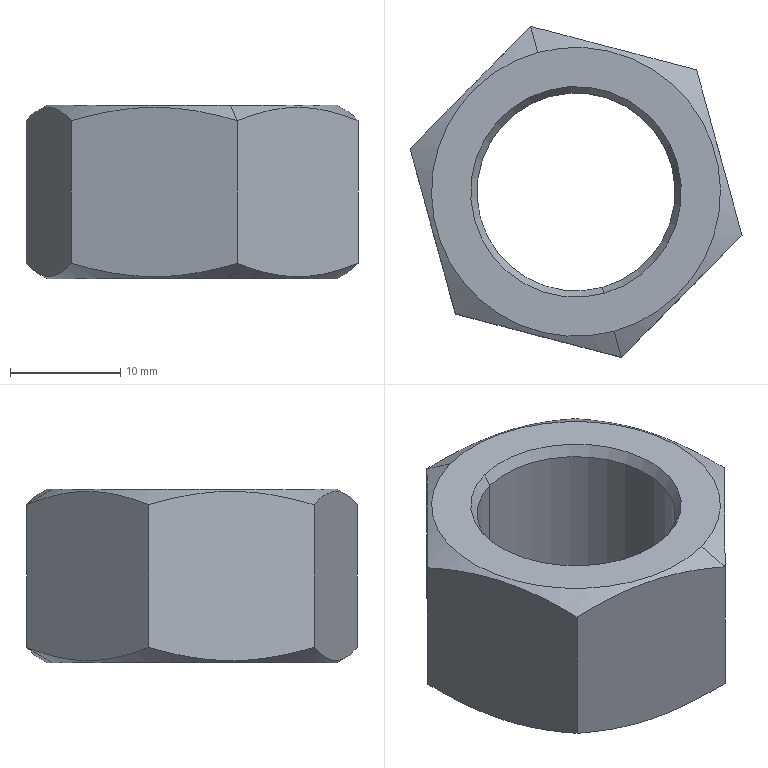Component | SolidWorks | Cylinder-1_hex nuts 1-fine pitch-grades ab gb-9 | 1 solid | 18 faces | box 30.16 x 30.07 x 15.8 mm | volume 5847 mm3 | cone 8 | plane 8 | cylinder 2 | commonest cylinder face diameters 18 x2
STEP:
#1=COLOUR_RGB('',0.7922,0.8196,0.9333);
#2=FILL_AREA_STYLE_COLOUR('',#1);
#3=FILL_AREA_STYLE('',(#2));
#4=SURFACE_STYLE_FILL_AREA(#3);
#5=SURFACE_SIDE_STYLE('',(#4));
#6=SURFACE_STYLE_USAGE(.BOTH.,#5);
#7=PRESENTATION_STYLE_ASSIGNMENT((#6));
#8=CARTESIAN_POINT('',(-7.202,1.382,-13.665));
#9=VERTEX_POINT('',#8);
#10=CARTESIAN_POINT('',(-7.015,0.6981,-13.665));
#11=VERTEX_POINT('',#10);
#12=CARTESIAN_POINT('',(-7.109,1.04,-13.665));
#13=DIRECTION('',(0.,-0.,-1.));
#14=DIRECTION('',(-0.2645,0.9644,0.));
#15=AXIS2_PLACEMENT_3D('',#12,#13,#14);
#16=CIRCLE('',#15,0.3543);
#17=EDGE_CURVE('',#9,#11,#16,.T.);
#18=ORIENTED_EDGE('',*,*,#17,.F.);
#19=CARTESIAN_POINT('',(-7.213,1.419,-13.687));
#20=VERTEX_POINT('',#19);
#21=CARTESIAN_POINT('',(-7.202,1.382,-13.665));
#22=DIRECTION('',(-0.2291,0.8352,-0.5));
#23=VECTOR('',#22,39.37);
#24=LINE('',#21,#23);
#25=EDGE_CURVE('',#9,#20,#24,.T.);
#26=ORIENTED_EDGE('',*,*,#25,.T.);
#27=CARTESIAN_POINT('',(-7.005,0.6606,-13.687));
#28=VERTEX_POINT('',#27);
#29=CARTESIAN_POINT('',(-7.109,1.04,-13.687));
#30=DIRECTION('',(-0.,0.,1.));
#31=DIRECTION('',(-0.2645,0.9644,0.));
#32=AXIS2_PLACEMENT_3D('',#29,#30,#31);
#33=CIRCLE('',#32,0.3932);
#34=EDGE_CURVE('',#28,#20,#33,.T.);
#35=ORIENTED_EDGE('',*,*,#34,.F.);
#36=CARTESIAN_POINT('',(-7.015,0.6981,-13.665));
#37=DIRECTION('',(0.2291,-0.8352,-0.5));
#38=VECTOR('',#37,39.37);
#39=LINE('',#36,#38);
#40=EDGE_CURVE('',#11,#28,#39,.T.);
#41=ORIENTED_EDGE('',*,*,#40,.F.);
#42=EDGE_LOOP('',(#18,#26,#35,#41));
#43=FACE_OUTER_BOUND('',#42,.T.);
#44=CARTESIAN_POINT('',(-7.109,1.04,-13.665));
#45=DIRECTION('',(0.,-0.,-1.));
#46=DIRECTION('',(0.2645,-0.9644,0.));
#47=AXIS2_PLACEMENT_3D('',#44,#45,#46);
#48=CONICAL_SURFACE('',#47,0.3543,1.047);
#49=ADVANCED_FACE('',(#43),#48,.F.);
#50=CARTESIAN_POINT('',(-7.015,0.6981,-13.104));
#51=VERTEX_POINT('',#50);
#52=CARTESIAN_POINT('',(-7.202,1.382,-13.104));
#53=VERTEX_POINT('',#52);
#54=CARTESIAN_POINT('',(-7.109,1.04,-13.104));
#55=DIRECTION('',(-0.,0.,1.));
#56=DIRECTION('',(-0.2645,0.9644,0.));
#57=AXIS2_PLACEMENT_3D('',#54,#55,#56);
#58=CIRCLE('',#57,0.3543);
#59=EDGE_CURVE('',#51,#53,#58,.T.);
#60=ORIENTED_EDGE('',*,*,#59,.F.);
#61=CARTESIAN_POINT('',(-7.009,0.6765,-13.065));
#62=VERTEX_POINT('',#61);
#63=CARTESIAN_POINT('',(-7.009,0.6765,-13.065));
#64=DIRECTION('',(0.1323,-0.4822,0.866));
#65=VECTOR('',#64,39.37);
#66=LINE('',#63,#65);
#67=EDGE_CURVE('',#51,#62,#66,.T.);
#68=ORIENTED_EDGE('',*,*,#67,.T.);
#69=CARTESIAN_POINT('',(-7.208,1.403,-13.065));
#70=VERTEX_POINT('',#69);
#71=CARTESIAN_POINT('',(-7.109,1.04,-13.065));
#72=DIRECTION('',(0.,-0.,-1.));
#73=DIRECTION('',(-0.2645,0.9644,0.));
#74=AXIS2_PLACEMENT_3D('',#71,#72,#73);
#75=CIRCLE('',#74,0.3768);
#76=EDGE_CURVE('',#70,#62,#75,.T.);
#77=ORIENTED_EDGE('',*,*,#76,.F.);
#78=CARTESIAN_POINT('',(-7.208,1.403,-13.065));
#79=DIRECTION('',(-0.1323,0.4822,0.866));
#80=VECTOR('',#79,39.37);
#81=LINE('',#78,#80);
#82=EDGE_CURVE('',#53,#70,#81,.T.);
#83=ORIENTED_EDGE('',*,*,#82,.F.);
#84=EDGE_LOOP('',(#60,#68,#77,#83));
#85=FACE_OUTER_BOUND('',#84,.T.);
#86=CARTESIAN_POINT('',(-7.109,1.04,-13.065));
#87=DIRECTION('',(-0.,0.,1.));
#88=DIRECTION('',(-0.2645,0.9644,0.));
#89=AXIS2_PLACEMENT_3D('',#86,#87,#88);
#90=CONICAL_SURFACE('',#89,0.3768,0.5236);
#91=ADVANCED_FACE('',(#85),#90,.F.);
#92=CARTESIAN_POINT('',(-7.245,1.538,-13.687));
#93=VERTEX_POINT('',#92);
#94=CARTESIAN_POINT('',(-6.972,0.5415,-13.687));
#95=VERTEX_POINT('',#94);
#96=CARTESIAN_POINT('',(-7.109,1.04,-13.687));
#97=DIRECTION('',(0.,0.,1.));
#98=DIRECTION('',(-0.2645,0.9644,0.));
#99=AXIS2_PLACEMENT_3D('',#96,#97,#98);
#100=CIRCLE('',#99,0.5167);
#101=EDGE_CURVE('',#93,#95,#100,.T.);
#102=ORIENTED_EDGE('',*,*,#101,.T.);
#103=CARTESIAN_POINT('',(-6.946,0.448,-13.631));
#104=VERTEX_POINT('',#103);
#105=CARTESIAN_POINT('',(-6.972,0.5415,-13.687));
#106=DIRECTION('',(0.2291,-0.8352,0.5));
#107=VECTOR('',#106,39.37);
#108=LINE('',#105,#107);
#109=EDGE_CURVE('',#95,#104,#108,.T.);
#110=ORIENTED_EDGE('',*,*,#109,.T.);
#111=CARTESIAN_POINT('',(-7.54,0.6033,-13.631));
#112=VERTEX_POINT('',#111);
#113=CARTESIAN_POINT('',(-6.946,0.448,-13.631));
#114=CARTESIAN_POINT('',(-6.995,0.4607,-13.646));
#115=CARTESIAN_POINT('',(-7.043,0.4734,-13.657));
#116=CARTESIAN_POINT('',(-7.142,0.4993,-13.674));
#117=CARTESIAN_POINT('',(-7.192,0.5123,-13.678));
#118=CARTESIAN_POINT('',(-7.268,0.5321,-13.679));
#119=CARTESIAN_POINT('',(-7.293,0.5387,-13.677));
#120=CARTESIAN_POINT('',(-7.343,0.5519,-13.673));
#121=CARTESIAN_POINT('',(-7.368,0.5584,-13.67));
#122=CARTESIAN_POINT('',(-7.442,0.5778,-13.657));
#123=CARTESIAN_POINT('',(-7.491,0.5906,-13.646));
#124=CARTESIAN_POINT('',(-7.54,0.6033,-13.631));
#125=B_SPLINE_CURVE_WITH_KNOTS('',3,(#113,#114,#115,#116,#117,#118,#119,#120,#121,#122,#123,#124),.UNSPECIFIED.,.F.,.F.,(4,2,2,2,2,4),(0.00000024,0.003936,0.007872,0.00984,0.01181,0.01574),.UNSPECIFIED.);
#126=EDGE_CURVE('',#104,#112,#125,.T.);
#127=ORIENTED_EDGE('',*,*,#126,.T.);
#128=CARTESIAN_POINT('',(-7.702,1.195,-13.631));
#129=VERTEX_POINT('',#128);
#130=CARTESIAN_POINT('',(-7.54,0.6033,-13.631));
#131=CARTESIAN_POINT('',(-7.553,0.6511,-13.645));
#132=CARTESIAN_POINT('',(-7.566,0.6996,-13.657));
#133=CARTESIAN_POINT('',(-7.587,0.7737,-13.67));
#134=CARTESIAN_POINT('',(-7.594,0.7987,-13.673));
#135=CARTESIAN_POINT('',(-7.607,0.8491,-13.677));
#136=CARTESIAN_POINT('',(-7.614,0.8741,-13.679));
#137=CARTESIAN_POINT('',(-7.635,0.9492,-13.679));
#138=CARTESIAN_POINT('',(-7.648,0.9989,-13.674));
#139=CARTESIAN_POINT('',(-7.669,1.073,-13.662));
#140=CARTESIAN_POINT('',(-7.676,1.098,-13.657));
#141=CARTESIAN_POINT('',(-7.689,1.147,-13.645));
#142=CARTESIAN_POINT('',(-7.696,1.171,-13.638));
#143=CARTESIAN_POINT('',(-7.702,1.195,-13.631));
#144=B_SPLINE_CURVE_WITH_KNOTS('',3,(#130,#131,#132,#133,#134,#135,#136,#137,#138,#139,#140,#141,#142,#143),.UNSPECIFIED.,.F.,.F.,(4,2,2,2,2,2,4),(0.005749,0.009683,0.01165,0.01362,0.01755,0.01952,0.02148),.UNSPECIFIED.);
#145=EDGE_CURVE('',#112,#129,#144,.T.);
#146=ORIENTED_EDGE('',*,*,#145,.T.);
#147=CARTESIAN_POINT('',(-7.271,1.632,-13.631));
#148=VERTEX_POINT('',#147);
#149=CARTESIAN_POINT('',(-7.702,1.195,-13.631));
#150=CARTESIAN_POINT('',(-7.667,1.231,-13.646));
#151=CARTESIAN_POINT('',(-7.632,1.267,-13.657));
#152=CARTESIAN_POINT('',(-7.56,1.339,-13.674));
#153=CARTESIAN_POINT('',(-7.524,1.376,-13.678));
#154=CARTESIAN_POINT('',(-7.469,1.432,-13.679));
#155=CARTESIAN_POINT('',(-7.45,1.45,-13.677));
#156=CARTESIAN_POINT('',(-7.414,1.487,-13.673));
#157=CARTESIAN_POINT('',(-7.396,1.505,-13.67));
#158=CARTESIAN_POINT('',(-7.342,1.56,-13.657));
#159=CARTESIAN_POINT('',(-7.306,1.596,-13.646));
#160=CARTESIAN_POINT('',(-7.271,1.632,-13.631));
#161=B_SPLINE_CURVE_WITH_KNOTS('',3,(#149,#150,#151,#152,#153,#154,#155,#156,#157,#158,#159,#160),.UNSPECIFIED.,.F.,.F.,(4,2,2,2,2,4),(0.00000024,0.003936,0.007872,0.00984,0.01181,0.01574),.UNSPECIFIED.);
#162=EDGE_CURVE('',#129,#148,#161,.T.);
#163=ORIENTED_EDGE('',*,*,#162,.T.);
#164=CARTESIAN_POINT('',(-7.245,1.538,-13.687));
#165=DIRECTION('',(-0.2291,0.8352,0.5));
#166=VECTOR('',#165,39.37);
#167=LINE('',#164,#166);
#168=EDGE_CURVE('',#93,#148,#167,.T.);
#169=ORIENTED_EDGE('',*,*,#168,.F.);
#170=EDGE_LOOP('',(#102,#110,#127,#146,#163,#169));
#171=FACE_OUTER_BOUND('',#170,.T.);
#172=CARTESIAN_POINT('',(-7.109,1.04,-13.687));
#173=DIRECTION('',(0.,0.,1.));
#174=DIRECTION('',(-0.2645,0.9644,0.));
#175=AXIS2_PLACEMENT_3D('',#172,#173,#174);
#176=CONICAL_SURFACE('',#175,0.5167,1.047);
#177=ADVANCED_FACE('',(#171),#176,.T.);
#178=CARTESIAN_POINT('',(-7.245,1.538,-13.065));
#179=VERTEX_POINT('',#178);
#180=CARTESIAN_POINT('',(-6.972,0.5415,-13.065));
#181=VERTEX_POINT('',#180);
#182=CARTESIAN_POINT('',(-7.109,1.04,-13.065));
#183=DIRECTION('',(0.,0.,1.));
#184=DIRECTION('',(-0.2645,0.9644,0.));
#185=AXIS2_PLACEMENT_3D('',#182,#183,#184);
#186=CIRCLE('',#185,0.5167);
#187=EDGE_CURVE('',#179,#181,#186,.T.);
#188=ORIENTED_EDGE('',*,*,#187,.F.);
#189=CARTESIAN_POINT('',(-7.271,1.632,-13.121));
#190=VERTEX_POINT('',#189);
#191=CARTESIAN_POINT('',(-7.271,1.632,-13.121));
#192=DIRECTION('',(-0.2291,0.8352,-0.5));
#193=VECTOR('',#192,39.37);
#194=LINE('',#191,#193);
#195=EDGE_CURVE('',#179,#190,#194,.T.);
#196=ORIENTED_EDGE('',*,*,#195,.T.);
#197=CARTESIAN_POINT('',(-7.702,1.195,-13.121));
#198=VERTEX_POINT('',#197);
#199=CARTESIAN_POINT('',(-7.271,1.632,-13.121));
#200=CARTESIAN_POINT('',(-7.306,1.596,-13.107));
#201=CARTESIAN_POINT('',(-7.342,1.56,-13.095));
#202=CARTESIAN_POINT('',(-7.413,1.488,-13.078));
#203=CARTESIAN_POINT('',(-7.449,1.451,-13.074));
#204=CARTESIAN_POINT('',(-7.505,1.395,-13.074));
#205=CARTESIAN_POINT('',(-7.523,1.377,-13.075));
#206=CARTESIAN_POINT('',(-7.559,1.34,-13.079));
#207=CARTESIAN_POINT('',(-7.577,1.321,-13.082));
#208=CARTESIAN_POINT('',(-7.631,1.267,-13.095));
#209=CARTESIAN_POINT('',(-7.667,1.231,-13.107));
#210=CARTESIAN_POINT('',(-7.702,1.195,-13.121));
#211=B_SPLINE_CURVE_WITH_KNOTS('',3,(#199,#200,#201,#202,#203,#204,#205,#206,#207,#208,#209,#210),.UNSPECIFIED.,.F.,.F.,(4,2,2,2,2,4),(0.00000024,0.003936,0.007872,0.00984,0.01181,0.01574),.UNSPECIFIED.);
#212=EDGE_CURVE('',#190,#198,#211,.T.);
#213=ORIENTED_EDGE('',*,*,#212,.T.);
#214=CARTESIAN_POINT('',(-7.54,0.6033,-13.121));
#215=VERTEX_POINT('',#214);
#216=CARTESIAN_POINT('',(-7.702,1.195,-13.121));
#217=CARTESIAN_POINT('',(-7.696,1.171,-13.114));
#218=CARTESIAN_POINT('',(-7.689,1.147,-13.107));
#219=CARTESIAN_POINT('',(-7.676,1.098,-13.095));
#220=CARTESIAN_POINT('',(-7.669,1.073,-13.09));
#221=CARTESIAN_POINT('',(-7.648,0.9989,-13.078));
#222=CARTESIAN_POINT('',(-7.635,0.9492,-13.074));
#223=CARTESIAN_POINT('',(-7.614,0.8741,-13.074));
#224=CARTESIAN_POINT('',(-7.607,0.8491,-13.075));
#225=CARTESIAN_POINT('',(-7.594,0.7987,-13.079));
#226=CARTESIAN_POINT('',(-7.587,0.7737,-13.082));
#227=CARTESIAN_POINT('',(-7.566,0.6996,-13.095));
#228=CARTESIAN_POINT('',(-7.553,0.6511,-13.107));
#229=CARTESIAN_POINT('',(-7.54,0.6033,-13.121));
#230=B_SPLINE_CURVE_WITH_KNOTS('',3,(#216,#217,#218,#219,#220,#221,#222,#223,#224,#225,#226,#227,#228,#229),.UNSPECIFIED.,.F.,.F.,(4,2,2,2,2,2,4),(0.01387,0.01584,0.01782,0.02176,0.02373,0.0257,0.02965),.UNSPECIFIED.);
#231=EDGE_CURVE('',#198,#215,#230,.T.);
#232=ORIENTED_EDGE('',*,*,#231,.T.);
#233=CARTESIAN_POINT('',(-6.946,0.448,-13.121));
#234=VERTEX_POINT('',#233);
#235=CARTESIAN_POINT('',(-7.54,0.6033,-13.121));
#236=CARTESIAN_POINT('',(-7.491,0.5906,-13.107));
#237=CARTESIAN_POINT('',(-7.443,0.5779,-13.095));
#238=CARTESIAN_POINT('',(-7.344,0.552,-13.078));
#239=CARTESIAN_POINT('',(-7.294,0.539,-13.074));
#240=CARTESIAN_POINT('',(-7.218,0.5192,-13.074));
#241=CARTESIAN_POINT('',(-7.193,0.5126,-13.075));
#242=CARTESIAN_POINT('',(-7.143,0.4994,-13.079));
#243=CARTESIAN_POINT('',(-7.118,0.4929,-13.082));
#244=CARTESIAN_POINT('',(-7.044,0.4735,-13.095));
#245=CARTESIAN_POINT('',(-6.995,0.4607,-13.107));
#246=CARTESIAN_POINT('',(-6.946,0.448,-13.121));
#247=B_SPLINE_CURVE_WITH_KNOTS('',3,(#235,#236,#237,#238,#239,#240,#241,#242,#243,#244,#245,#246),.UNSPECIFIED.,.F.,.F.,(4,2,2,2,2,4),(0.00000024,0.003936,0.007872,0.00984,0.01181,0.01574),.UNSPECIFIED.);
#248=EDGE_CURVE('',#215,#234,#247,.T.);
#249=ORIENTED_EDGE('',*,*,#248,.T.);
#250=CARTESIAN_POINT('',(-6.946,0.448,-13.121));
#251=DIRECTION('',(0.2291,-0.8352,-0.5));
#252=VECTOR('',#251,39.37);
#253=LINE('',#250,#252);
#254=EDGE_CURVE('',#181,#234,#253,.T.);
#255=ORIENTED_EDGE('',*,*,#254,.F.);
#256=EDGE_LOOP('',(#188,#196,#213,#232,#249,#255));
#257=FACE_OUTER_BOUND('',#256,.T.);
#258=CARTESIAN_POINT('',(-7.109,1.04,-13.121));
#259=DIRECTION('',(-0.,-0.,-1.));
#260=DIRECTION('',(0.2645,-0.9644,0.));
#261=AXIS2_PLACEMENT_3D('',#258,#259,#260);
#262=CONICAL_SURFACE('',#261,0.6137,1.047);
#263=ADVANCED_FACE('',(#257),#262,.T.);
#264=ORIENTED_EDGE('',*,*,#59,.T.);
#265=CARTESIAN_POINT('',(-7.202,1.382,-13.065));
#266=DIRECTION('',(0.,-0.,-1.));
#267=VECTOR('',#266,39.37);
#268=LINE('',#265,#267);
#269=EDGE_CURVE('',#53,#9,#268,.T.);
#270=ORIENTED_EDGE('',*,*,#269,.T.);
#271=ORIENTED_EDGE('',*,*,#17,.T.);
#272=CARTESIAN_POINT('',(-7.015,0.6981,-13.065));
#273=DIRECTION('',(0.,-0.,-1.));
#274=VECTOR('',#273,39.37);
#275=LINE('',#272,#274);
#276=EDGE_CURVE('',#51,#11,#275,.T.);
#277=ORIENTED_EDGE('',*,*,#276,.F.);
#278=EDGE_LOOP('',(#264,#270,#271,#277));
#279=FACE_OUTER_BOUND('',#278,.T.);
#280=CARTESIAN_POINT('',(-7.109,1.04,-13.065));
#281=DIRECTION('',(0.,-0.,-1.));
#282=DIRECTION('',(0.2645,-0.9644,0.));
#283=AXIS2_PLACEMENT_3D('',#280,#281,#282);
#284=CYLINDRICAL_SURFACE('',#283,0.3543);
#285=ADVANCED_FACE('',(#279),#284,.F.);
#286=CARTESIAN_POINT('',(-6.677,1.476,-13.631));
#287=VERTEX_POINT('',#286);
#288=CARTESIAN_POINT('',(-6.515,0.8845,-13.631));
#289=VERTEX_POINT('',#288);
#290=CARTESIAN_POINT('',(-6.677,1.476,-13.631));
#291=CARTESIAN_POINT('',(-6.671,1.452,-13.638));
#292=CARTESIAN_POINT('',(-6.664,1.428,-13.645));
#293=CARTESIAN_POINT('',(-6.65,1.379,-13.657));
#294=CARTESIAN_POINT('',(-6.644,1.354,-13.662));
#295=CARTESIAN_POINT('',(-6.623,1.28,-13.674));
#296=CARTESIAN_POINT('',(-6.61,1.23,-13.679));
#297=CARTESIAN_POINT('',(-6.589,1.155,-13.679));
#298=CARTESIAN_POINT('',(-6.582,1.13,-13.677));
#299=CARTESIAN_POINT('',(-6.568,1.08,-13.673));
#300=CARTESIAN_POINT('',(-6.562,1.055,-13.67));
#301=CARTESIAN_POINT('',(-6.541,0.9808,-13.657));
#302=CARTESIAN_POINT('',(-6.528,0.9323,-13.645));
#303=CARTESIAN_POINT('',(-6.515,0.8845,-13.631));
#304=B_SPLINE_CURVE_WITH_KNOTS('',3,(#290,#291,#292,#293,#294,#295,#296,#297,#298,#299,#300,#301,#302,#303),.UNSPECIFIED.,.F.,.F.,(4,2,2,2,2,2,4),(0.01387,0.01584,0.01782,0.02176,0.02373,0.0257,0.02965),.UNSPECIFIED.);
#305=EDGE_CURVE('',#287,#289,#304,.T.);
#306=ORIENTED_EDGE('',*,*,#305,.F.);
#307=CARTESIAN_POINT('',(-6.677,1.476,-13.121));
#308=VERTEX_POINT('',#307);
#309=CARTESIAN_POINT('',(-6.677,1.476,-13.065));
#310=DIRECTION('',(0.,-0.,-1.));
#311=VECTOR('',#310,39.37);
#312=LINE('',#309,#311);
#313=EDGE_CURVE('',#308,#287,#312,.T.);
#314=ORIENTED_EDGE('',*,*,#313,.F.);
#315=CARTESIAN_POINT('',(-6.515,0.8845,-13.121));
#316=VERTEX_POINT('',#315);
#317=CARTESIAN_POINT('',(-6.515,0.8845,-13.121));
#318=CARTESIAN_POINT('',(-6.528,0.9323,-13.107));
#319=CARTESIAN_POINT('',(-6.541,0.9808,-13.095));
#320=CARTESIAN_POINT('',(-6.562,1.055,-13.082));
#321=CARTESIAN_POINT('',(-6.568,1.08,-13.079));
#322=CARTESIAN_POINT('',(-6.582,1.13,-13.075));
#323=CARTESIAN_POINT('',(-6.589,1.155,-13.074));
#324=CARTESIAN_POINT('',(-6.61,1.23,-13.074));
#325=CARTESIAN_POINT('',(-6.623,1.28,-13.078));
#326=CARTESIAN_POINT('',(-6.644,1.354,-13.09));
#327=CARTESIAN_POINT('',(-6.65,1.379,-13.095));
#328=CARTESIAN_POINT('',(-6.664,1.428,-13.107));
#329=CARTESIAN_POINT('',(-6.671,1.452,-13.114));
#330=CARTESIAN_POINT('',(-6.677,1.476,-13.121));
#331=B_SPLINE_CURVE_WITH_KNOTS('',3,(#317,#318,#319,#320,#321,#322,#323,#324,#325,#326,#327,#328,#329,#330),.UNSPECIFIED.,.F.,.F.,(4,2,2,2,2,2,4),(0.005749,0.009683,0.01165,0.01362,0.01755,0.01952,0.02148),.UNSPECIFIED.);
#332=EDGE_CURVE('',#316,#308,#331,.T.);
#333=ORIENTED_EDGE('',*,*,#332,.F.);
#334=CARTESIAN_POINT('',(-6.515,0.8845,-13.065));
#335=DIRECTION('',(0.,-0.,-1.));
#336=VECTOR('',#335,39.37);
#337=LINE('',#334,#336);
#338=EDGE_CURVE('',#316,#289,#337,.T.);
#339=ORIENTED_EDGE('',*,*,#338,.T.);
#340=EDGE_LOOP('',(#306,#314,#333,#339));
#341=FACE_OUTER_BOUND('',#340,.T.);
#342=CARTESIAN_POINT('',(-6.677,1.476,-13.065));
#343=DIRECTION('',(0.9644,0.2645,-0.));
#344=DIRECTION('',(0.2645,-0.9644,0.));
#345=AXIS2_PLACEMENT_3D('',#342,#343,#344);
#346=PLANE('',#345);
#347=ADVANCED_FACE('',(#341),#346,.T.);
#348=CARTESIAN_POINT('',(-7.271,1.632,-13.631));
#349=CARTESIAN_POINT('',(-7.222,1.619,-13.646));
#350=CARTESIAN_POINT('',(-7.174,1.606,-13.657));
#351=CARTESIAN_POINT('',(-7.075,1.58,-13.674));
#352=CARTESIAN_POINT('',(-7.025,1.567,-13.678));
#353=CARTESIAN_POINT('',(-6.949,1.548,-13.679));
#354=CARTESIAN_POINT('',(-6.924,1.541,-13.677));
#355=CARTESIAN_POINT('',(-6.874,1.528,-13.673));
#356=CARTESIAN_POINT('',(-6.849,1.521,-13.67));
#357=CARTESIAN_POINT('',(-6.775,1.502,-13.657));
#358=CARTESIAN_POINT('',(-6.726,1.489,-13.646));
#359=CARTESIAN_POINT('',(-6.677,1.476,-13.631));
#360=B_SPLINE_CURVE_WITH_KNOTS('',3,(#348,#349,#350,#351,#352,#353,#354,#355,#356,#357,#358,#359),.UNSPECIFIED.,.F.,.F.,(4,2,2,2,2,4),(0.00000024,0.003936,0.007872,0.00984,0.01181,0.01574),.UNSPECIFIED.);
#361=EDGE_CURVE('',#148,#287,#360,.T.);
#362=ORIENTED_EDGE('',*,*,#361,.F.);
#363=CARTESIAN_POINT('',(-7.271,1.632,-13.065));
#364=DIRECTION('',(0.,-0.,-1.));
#365=VECTOR('',#364,39.37);
#366=LINE('',#363,#365);
#367=EDGE_CURVE('',#190,#148,#366,.T.);
#368=ORIENTED_EDGE('',*,*,#367,.F.);
#369=CARTESIAN_POINT('',(-6.677,1.476,-13.121));
#370=CARTESIAN_POINT('',(-6.726,1.489,-13.107));
#371=CARTESIAN_POINT('',(-6.774,1.502,-13.095));
#372=CARTESIAN_POINT('',(-6.873,1.528,-13.078));
#373=CARTESIAN_POINT('',(-6.923,1.541,-13.074));
#374=CARTESIAN_POINT('',(-6.999,1.56,-13.074));
#375=CARTESIAN_POINT('',(-7.024,1.567,-13.075));
#376=CARTESIAN_POINT('',(-7.074,1.58,-13.079));
#377=CARTESIAN_POINT('',(-7.099,1.587,-13.082));
#378=CARTESIAN_POINT('',(-7.173,1.606,-13.095));
#379=CARTESIAN_POINT('',(-7.222,1.619,-13.107));
#380=CARTESIAN_POINT('',(-7.271,1.632,-13.121));
#381=B_SPLINE_CURVE_WITH_KNOTS('',3,(#369,#370,#371,#372,#373,#374,#375,#376,#377,#378,#379,#380),.UNSPECIFIED.,.F.,.F.,(4,2,2,2,2,4),(0.00000024,0.003936,0.007872,0.00984,0.01181,0.01574),.UNSPECIFIED.);
#382=EDGE_CURVE('',#308,#190,#381,.T.);
#383=ORIENTED_EDGE('',*,*,#382,.F.);
#384=ORIENTED_EDGE('',*,*,#313,.T.);
#385=EDGE_LOOP('',(#362,#368,#383,#384));
#386=FACE_OUTER_BOUND('',#385,.T.);
#387=CARTESIAN_POINT('',(-7.271,1.632,-13.065));
#388=DIRECTION('',(0.2531,0.9674,-0.));
#389=DIRECTION('',(0.9674,-0.2531,0.));
#390=AXIS2_PLACEMENT_3D('',#387,#388,#389);
#391=PLANE('',#390);
#392=ADVANCED_FACE('',(#386),#391,.T.);
#393=ORIENTED_EDGE('',*,*,#162,.F.);
#394=CARTESIAN_POINT('',(-7.702,1.195,-13.065));
#395=DIRECTION('',(0.,-0.,-1.));
#396=VECTOR('',#395,39.37);
#397=LINE('',#394,#396);
#398=EDGE_CURVE('',#198,#129,#397,.T.);
#399=ORIENTED_EDGE('',*,*,#398,.F.);
#400=ORIENTED_EDGE('',*,*,#212,.F.);
#401=ORIENTED_EDGE('',*,*,#367,.T.);
#402=EDGE_LOOP('',(#393,#399,#400,#401));
#403=FACE_OUTER_BOUND('',#402,.T.);
#404=CARTESIAN_POINT('',(-7.702,1.195,-13.065));
#405=DIRECTION('',(-0.7113,0.7029,-0.));
#406=DIRECTION('',(0.7029,0.7113,-0.));
#407=AXIS2_PLACEMENT_3D('',#404,#405,#406);
#408=PLANE('',#407);
#409=ADVANCED_FACE('',(#403),#408,.T.);
#410=ORIENTED_EDGE('',*,*,#145,.F.);
#411=CARTESIAN_POINT('',(-7.54,0.6033,-13.065));
#412=DIRECTION('',(0.,-0.,-1.));
#413=VECTOR('',#412,39.37);
#414=LINE('',#411,#413);
#415=EDGE_CURVE('',#215,#112,#414,.T.);
#416=ORIENTED_EDGE('',*,*,#415,.F.);
#417=ORIENTED_EDGE('',*,*,#231,.F.);
#418=ORIENTED_EDGE('',*,*,#398,.T.);
#419=EDGE_LOOP('',(#410,#416,#417,#418));
#420=FACE_OUTER_BOUND('',#419,.T.);
#421=CARTESIAN_POINT('',(-7.54,0.6033,-13.065));
#422=DIRECTION('',(-0.9644,-0.2645,0.));
#423=DIRECTION('',(0.,-0.,-1.));
#424=AXIS2_PLACEMENT_3D('',#421,#422,#423);
#425=PLANE('',#424);
#426=ADVANCED_FACE('',(#420),#425,.T.);
#427=ORIENTED_EDGE('',*,*,#126,.F.);
#428=CARTESIAN_POINT('',(-6.946,0.448,-13.065));
#429=DIRECTION('',(0.,-0.,-1.));
#430=VECTOR('',#429,39.37);
#431=LINE('',#428,#430);
#432=EDGE_CURVE('',#234,#104,#431,.T.);
#433=ORIENTED_EDGE('',*,*,#432,.F.);
#434=ORIENTED_EDGE('',*,*,#248,.F.);
#435=ORIENTED_EDGE('',*,*,#415,.T.);
#436=EDGE_LOOP('',(#427,#433,#434,#435));
#437=FACE_OUTER_BOUND('',#436,.T.);
#438=CARTESIAN_POINT('',(-6.946,0.448,-13.065));
#439=DIRECTION('',(-0.2531,-0.9674,0.));
#440=DIRECTION('',(-0.9674,0.2531,-0.));
#441=AXIS2_PLACEMENT_3D('',#438,#439,#440);
#442=PLANE('',#441);
#443=ADVANCED_FACE('',(#437),#442,.T.);
#444=CARTESIAN_POINT('',(-6.515,0.8845,-13.631));
#445=CARTESIAN_POINT('',(-6.55,0.8489,-13.646));
#446=CARTESIAN_POINT('',(-6.585,0.813,-13.657));
#447=CARTESIAN_POINT('',(-6.657,0.7404,-13.674));
#448=CARTESIAN_POINT('',(-6.693,0.7038,-13.678));
#449=CARTESIAN_POINT('',(-6.748,0.6481,-13.679));
#450=CARTESIAN_POINT('',(-6.767,0.6295,-13.677));
#451=CARTESIAN_POINT('',(-6.803,0.5926,-13.673));
#452=CARTESIAN_POINT('',(-6.821,0.5743,-13.67));
#453=CARTESIAN_POINT('',(-6.875,0.5196,-13.657));
#454=CARTESIAN_POINT('',(-6.911,0.4837,-13.646));
#455=CARTESIAN_POINT('',(-6.946,0.448,-13.631));
#456=B_SPLINE_CURVE_WITH_KNOTS('',3,(#444,#445,#446,#447,#448,#449,#450,#451,#452,#453,#454,#455),.UNSPECIFIED.,.F.,.F.,(4,2,2,2,2,4),(0.00000024,0.003936,0.007872,0.00984,0.01181,0.01574),.UNSPECIFIED.);
#457=EDGE_CURVE('',#289,#104,#456,.T.);
#458=ORIENTED_EDGE('',*,*,#457,.F.);
#459=ORIENTED_EDGE('',*,*,#338,.F.);
#460=CARTESIAN_POINT('',(-6.946,0.448,-13.121));
#461=CARTESIAN_POINT('',(-6.911,0.4836,-13.107));
#462=CARTESIAN_POINT('',(-6.875,0.5195,-13.095));
#463=CARTESIAN_POINT('',(-6.804,0.5921,-13.078));
#464=CARTESIAN_POINT('',(-6.768,0.6287,-13.074));
#465=CARTESIAN_POINT('',(-6.713,0.6844,-13.074));
#466=CARTESIAN_POINT('',(-6.694,0.703,-13.075));
#467=CARTESIAN_POINT('',(-6.658,0.7399,-13.079));
#468=CARTESIAN_POINT('',(-6.64,0.7582,-13.082));
#469=CARTESIAN_POINT('',(-6.586,0.8128,-13.095));
#470=CARTESIAN_POINT('',(-6.55,0.8488,-13.107));
#471=CARTESIAN_POINT('',(-6.515,0.8845,-13.121));
#472=B_SPLINE_CURVE_WITH_KNOTS('',3,(#460,#461,#462,#463,#464,#465,#466,#467,#468,#469,#470,#471),.UNSPECIFIED.,.F.,.F.,(4,2,2,2,2,4),(0.00000024,0.003936,0.007872,0.00984,0.01181,0.01574),.UNSPECIFIED.);
#473=EDGE_CURVE('',#234,#316,#472,.T.);
#474=ORIENTED_EDGE('',*,*,#473,.F.);
#475=ORIENTED_EDGE('',*,*,#432,.T.);
#476=EDGE_LOOP('',(#458,#459,#474,#475));
#477=FACE_OUTER_BOUND('',#476,.T.);
#478=CARTESIAN_POINT('',(-6.515,0.8845,-13.065));
#479=DIRECTION('',(0.7113,-0.7029,0.));
#480=DIRECTION('',(-0.7029,-0.7113,0.));
#481=AXIS2_PLACEMENT_3D('',#478,#479,#480);
#482=PLANE('',#481);
#483=ADVANCED_FACE('',(#477),#482,.T.);
#484=ORIENTED_EDGE('',*,*,#76,.T.);
#485=CARTESIAN_POINT('',(-7.109,1.04,-13.065));
#486=DIRECTION('',(0.,-0.,-1.));
#487=DIRECTION('',(-0.2645,0.9644,0.));
#488=AXIS2_PLACEMENT_3D('',#485,#486,#487);
#489=CIRCLE('',#488,0.3768);
#490=EDGE_CURVE('',#62,#70,#489,.T.);
#491=ORIENTED_EDGE('',*,*,#490,.T.);
#492=EDGE_LOOP('',(#484,#491));
#493=FACE_BOUND('',#492,.T.);
#494=CARTESIAN_POINT('',(-7.109,1.04,-13.065));
#495=DIRECTION('',(0.,0.,1.));
#496=DIRECTION('',(-0.2645,0.9644,0.));
#497=AXIS2_PLACEMENT_3D('',#494,#495,#496);
#498=CIRCLE('',#497,0.5167);
#499=EDGE_CURVE('',#181,#179,#498,.T.);
#500=ORIENTED_EDGE('',*,*,#499,.T.);
#501=ORIENTED_EDGE('',*,*,#187,.T.);
#502=EDGE_LOOP('',(#500,#501));
#503=FACE_OUTER_BOUND('',#502,.T.);
#504=CARTESIAN_POINT('',(-6.677,1.476,-13.065));
#505=DIRECTION('',(-0.,0.,1.));
#506=DIRECTION('',(-0.2645,0.9644,-0.));
#507=AXIS2_PLACEMENT_3D('',#504,#505,#506);
#508=PLANE('',#507);
#509=ADVANCED_FACE('',(#493,#503),#508,.T.);
#510=ORIENTED_EDGE('',*,*,#34,.T.);
#511=CARTESIAN_POINT('',(-7.109,1.04,-13.687));
#512=DIRECTION('',(-0.,0.,1.));
#513=DIRECTION('',(-0.2645,0.9644,0.));
#514=AXIS2_PLACEMENT_3D('',#511,#512,#513);
#515=CIRCLE('',#514,0.3932);
#516=EDGE_CURVE('',#20,#28,#515,.T.);
#517=ORIENTED_EDGE('',*,*,#516,.T.);
#518=EDGE_LOOP('',(#510,#517));
#519=FACE_BOUND('',#518,.T.);
#520=ORIENTED_EDGE('',*,*,#101,.F.);
#521=CARTESIAN_POINT('',(-7.109,1.04,-13.687));
#522=DIRECTION('',(0.,0.,1.));
#523=DIRECTION('',(-0.2645,0.9644,0.));
#524=AXIS2_PLACEMENT_3D('',#521,#522,#523);
#525=CIRCLE('',#524,0.5167);
#526=EDGE_CURVE('',#95,#93,#525,.T.);
#527=ORIENTED_EDGE('',*,*,#526,.F.);
#528=EDGE_LOOP('',(#520,#527));
#529=FACE_OUTER_BOUND('',#528,.T.);
#530=CARTESIAN_POINT('',(-6.677,1.476,-13.687));
#531=DIRECTION('',(-0.,0.,1.));
#532=DIRECTION('',(-0.2645,0.9644,-0.));
#533=AXIS2_PLACEMENT_3D('',#530,#531,#532);
#534=PLANE('',#533);
#535=ADVANCED_FACE('',(#519,#529),#534,.F.);
#536=ORIENTED_EDGE('',*,*,#269,.F.);
#537=CARTESIAN_POINT('',(-7.109,1.04,-13.104));
#538=DIRECTION('',(-0.,0.,1.));
#539=DIRECTION('',(-0.2645,0.9644,0.));
#540=AXIS2_PLACEMENT_3D('',#537,#538,#539);
#541=CIRCLE('',#540,0.3543);
#542=EDGE_CURVE('',#53,#51,#541,.T.);
#543=ORIENTED_EDGE('',*,*,#542,.T.);
#544=ORIENTED_EDGE('',*,*,#276,.T.);
#545=CARTESIAN_POINT('',(-7.109,1.04,-13.665));
#546=DIRECTION('',(0.,-0.,-1.));
#547=DIRECTION('',(-0.2645,0.9644,0.));
#548=AXIS2_PLACEMENT_3D('',#545,#546,#547);
#549=CIRCLE('',#548,0.3543);
#550=EDGE_CURVE('',#11,#9,#549,.T.);
#551=ORIENTED_EDGE('',*,*,#550,.T.);
#552=EDGE_LOOP('',(#536,#543,#544,#551));
#553=FACE_OUTER_BOUND('',#552,.T.);
#554=CARTESIAN_POINT('',(-7.109,1.04,-13.065));
#555=DIRECTION('',(0.,-0.,-1.));
#556=DIRECTION('',(0.2645,-0.9644,0.));
#557=AXIS2_PLACEMENT_3D('',#554,#555,#556);
#558=CYLINDRICAL_SURFACE('',#557,0.3543);
#559=ADVANCED_FACE('',(#553),#558,.F.);
#560=ORIENTED_EDGE('',*,*,#195,.F.);
#561=ORIENTED_EDGE('',*,*,#499,.F.);
#562=ORIENTED_EDGE('',*,*,#254,.T.);
#563=ORIENTED_EDGE('',*,*,#473,.T.);
#564=ORIENTED_EDGE('',*,*,#332,.T.);
#565=ORIENTED_EDGE('',*,*,#382,.T.);
#566=EDGE_LOOP('',(#560,#561,#562,#563,#564,#565));
#567=FACE_OUTER_BOUND('',#566,.T.);
#568=CARTESIAN_POINT('',(-7.109,1.04,-13.121));
#569=DIRECTION('',(-0.,-0.,-1.));
#570=DIRECTION('',(0.2645,-0.9644,0.));
#571=AXIS2_PLACEMENT_3D('',#568,#569,#570);
#572=CONICAL_SURFACE('',#571,0.6137,1.047);
#573=ADVANCED_FACE('',(#567),#572,.T.);
#574=ORIENTED_EDGE('',*,*,#109,.F.);
#575=ORIENTED_EDGE('',*,*,#526,.T.);
#576=ORIENTED_EDGE('',*,*,#168,.T.);
#577=ORIENTED_EDGE('',*,*,#361,.T.);
#578=ORIENTED_EDGE('',*,*,#305,.T.);
#579=ORIENTED_EDGE('',*,*,#457,.T.);
#580=EDGE_LOOP('',(#574,#575,#576,#577,#578,#579));
#581=FACE_OUTER_BOUND('',#580,.T.);
#582=CARTESIAN_POINT('',(-7.109,1.04,-13.687));
#583=DIRECTION('',(0.,0.,1.));
#584=DIRECTION('',(-0.2645,0.9644,0.));
#585=AXIS2_PLACEMENT_3D('',#582,#583,#584);
#586=CONICAL_SURFACE('',#585,0.5167,1.047);
#587=ADVANCED_FACE('',(#581),#586,.T.);
#588=ORIENTED_EDGE('',*,*,#67,.F.);
#589=ORIENTED_EDGE('',*,*,#542,.F.);
#590=ORIENTED_EDGE('',*,*,#82,.T.);
#591=ORIENTED_EDGE('',*,*,#490,.F.);
#592=EDGE_LOOP('',(#588,#589,#590,#591));
#593=FACE_OUTER_BOUND('',#592,.T.);
#594=CARTESIAN_POINT('',(-7.109,1.04,-13.065));
#595=DIRECTION('',(-0.,0.,1.));
#596=DIRECTION('',(-0.2645,0.9644,0.));
#597=AXIS2_PLACEMENT_3D('',#594,#595,#596);
#598=CONICAL_SURFACE('',#597,0.3768,0.5236);
#599=ADVANCED_FACE('',(#593),#598,.F.);
#600=ORIENTED_EDGE('',*,*,#25,.F.);
#601=ORIENTED_EDGE('',*,*,#550,.F.);
#602=ORIENTED_EDGE('',*,*,#40,.T.);
#603=ORIENTED_EDGE('',*,*,#516,.F.);
#604=EDGE_LOOP('',(#600,#601,#602,#603));
#605=FACE_OUTER_BOUND('',#604,.T.);
#606=CARTESIAN_POINT('',(-7.109,1.04,-13.665));
#607=DIRECTION('',(0.,-0.,-1.));
#608=DIRECTION('',(0.2645,-0.9644,0.));
#609=AXIS2_PLACEMENT_3D('',#606,#607,#608);
#610=CONICAL_SURFACE('',#609,0.3543,1.047);
#611=ADVANCED_FACE('',(#605),#610,.F.);
#612=CLOSED_SHELL('',(#49,#91,#177,#263,#285,#347,#392,#409,#426,#443,#483,#509,#535,#559,#573,#587,#599,#611));
#613=MANIFOLD_SOLID_BREP('',#612);
#614=STYLED_ITEM('',(#7),#613);
#615=PRESENTATION_LAYER_ASSIGNMENT('','',(#614));
#616=(LENGTH_UNIT()NAMED_UNIT(*)SI_UNIT($,.METRE.));
#617=LENGTH_MEASURE_WITH_UNIT(LENGTH_MEASURE(0.0254),#616);
#618=DIMENSIONAL_EXPONENTS(1.,0.,0.,0.,0.,0.,0.);
#619=(CONVERSION_BASED_UNIT('',#617)LENGTH_UNIT()NAMED_UNIT(#618));
#620=UNCERTAINTY_MEASURE_WITH_UNIT(LENGTH_MEASURE(0.00001),#619,'','');
#621=(NAMED_UNIT(*)PLANE_ANGLE_UNIT()SI_UNIT($,.RADIAN.));
#622=(NAMED_UNIT(*)SI_UNIT($,.STERADIAN.)SOLID_ANGLE_UNIT());
#623=(GEOMETRIC_REPRESENTATION_CONTEXT(3)GLOBAL_UNCERTAINTY_ASSIGNED_CONTEXT((#620))GLOBAL_UNIT_ASSIGNED_CONTEXT((#619,#621,#622))REPRESENTATION_CONTEXT('',''));
#624=MECHANICAL_DESIGN_GEOMETRIC_PRESENTATION_REPRESENTATION('',(#614),#623);
#625=CARTESIAN_POINT('',(0.,0.,0.));
#626=DIRECTION('',(0.,0.,1.));
#627=DIRECTION('',(1.,0.,0.));
#628=AXIS2_PLACEMENT_3D('',#625,#626,#627);
#629=(LENGTH_UNIT()NAMED_UNIT(*)SI_UNIT($,.METRE.));
#630=LENGTH_MEASURE_WITH_UNIT(LENGTH_MEASURE(0.0254),#629);
#631=DIMENSIONAL_EXPONENTS(1.,0.,0.,0.,0.,0.,0.);
#632=(CONVERSION_BASED_UNIT('',#630)LENGTH_UNIT()NAMED_UNIT(#631));
#633=UNCERTAINTY_MEASURE_WITH_UNIT(LENGTH_MEASURE(0.00001),#632,'','');
#634=(NAMED_UNIT(*)PLANE_ANGLE_UNIT()SI_UNIT($,.RADIAN.));
#635=(NAMED_UNIT(*)SI_UNIT($,.STERADIAN.)SOLID_ANGLE_UNIT());
#636=(GEOMETRIC_REPRESENTATION_CONTEXT(3)GLOBAL_UNCERTAINTY_ASSIGNED_CONTEXT((#633))GLOBAL_UNIT_ASSIGNED_CONTEXT((#632,#634,#635))REPRESENTATION_CONTEXT('',''));
#637=ADVANCED_BREP_SHAPE_REPRESENTATION('',(#613,#628),#636);